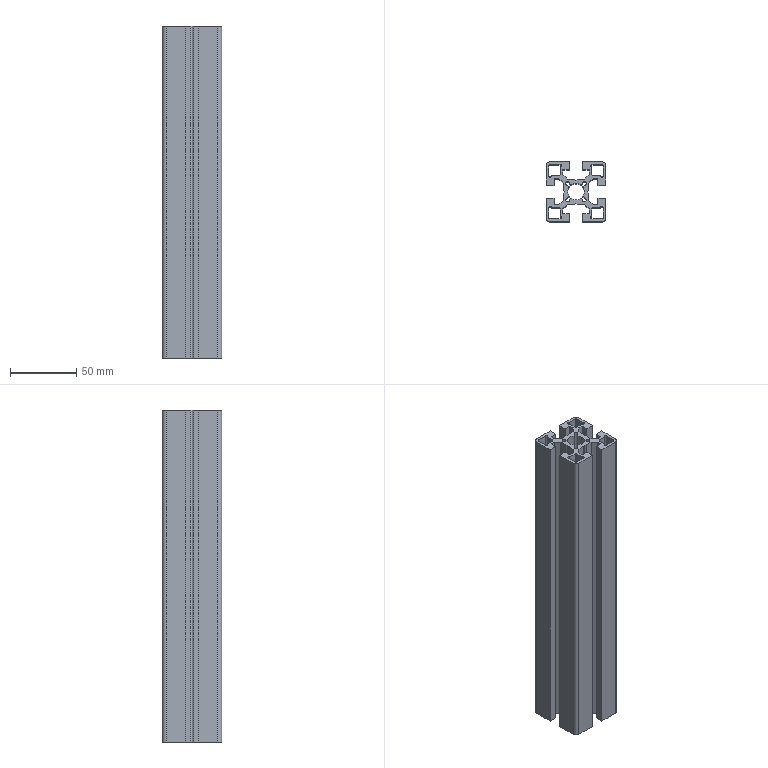Component | SolidWorks | HFS8_4545_08-B-3 | 1 solid | 131 faces | box 45 x 45 x 250 mm | volume 200550 mm3 | plane 82 | cylinder 49 | commonest cylinder face diameters 2 x18 3 x12 1 x10 12.5 x5 6 x4 | material 6061-T6 (SS)
build123d program:
from build123d import *

# Parameters (mm, degrees)
BOSS_EXTRUDE1_DEPTH = 250


with BuildPart() as part:
    # Sketch1 → Boss-Extrude1 (new body)
    with BuildSketch(Plane.XY):
        with BuildLine():
            Line((-19.5, -22.5), (-5, -22.5))
            Line((-5, -22.5), (-5, -16.5))
            Line((-5, -16.5), (-10, -16.5))
            Line((-10, -16.5), (-10, -13))
            Line((-10, -13), (-6.5, -9.5))
            Line((-6.5, -9.5), (-1.212, -9.5))
            Line((-1.212, -9.5), (0, -8.8))
            Line((0, -8.8), (1.212, -9.5))
            Line((1.212, -9.5), (6.5, -9.5))
            Line((6.5, -9.5), (10, -13))
            Line((10, -13), (10, -16.5))
            Line((10, -16.5), (5, -16.5))
            Line((5, -16.5), (5, -22.5))
            Line((5, -22.5), (19.5, -22.5))
            ThreePointArc((19.5, -22.5), (21.621, -21.621), (22.5, -19.5))
            Line((22.5, -19.5), (22.5, -5))
            Line((22.5, -5), (16.5, -5))
            Line((16.5, -5), (16.5, -10))
            Line((16.5, -10), (13, -10))
            Line((13, -10), (9.5, -6.5))
            Line((9.5, -6.5), (9.5, -1.212))
            Line((9.5, -1.212), (8.8, 0))
            Line((8.8, 0), (9.5, 1.212))
            Line((9.5, 1.212), (9.5, 6.5))
            Line((9.5, 6.5), (13, 10))
            Line((13, 10), (16.5, 10))
            Line((16.5, 10), (16.5, 5))
            Line((16.5, 5), (22.5, 5))
            Line((22.5, 5), (22.5, 19.5))
            ThreePointArc((22.5, 19.5), (21.621, 21.621), (19.5, 22.5))
            Line((19.5, 22.5), (5, 22.5))
            Line((5, 22.5), (5, 16.5))
            Line((5, 16.5), (10, 16.5))
            Line((10, 16.5), (10, 13))
            Line((10, 13), (6.5, 9.5))
            Line((6.5, 9.5), (1.212, 9.5))
            Line((1.212, 9.5), (0, 8.8))
            Line((0, 8.8), (-1.212, 9.5))
            Line((-1.212, 9.5), (-6.5, 9.5))
            Line((-6.5, 9.5), (-10, 13))
            Line((-10, 13), (-10, 16.5))
            Line((-10, 16.5), (-5, 16.5))
            Line((-5, 16.5), (-5, 22.5))
            Line((-5, 22.5), (-19.5, 22.5))
            ThreePointArc((-19.5, 22.5), (-21.621, 21.621), (-22.5, 19.5))
            Line((-22.5, 19.5), (-22.5, 5))
            Line((-22.5, 5), (-16.5, 5))
            Line((-16.5, 5), (-16.5, 10))
            Line((-16.5, 10), (-13, 10))
            Line((-13, 10), (-9.5, 6.5))
            Line((-9.5, 6.5), (-9.5, 1.212))
            Line((-9.5, 1.212), (-8.8, 0))
            Line((-8.8, 0), (-9.5, -1.212))
            Line((-9.5, -1.212), (-9.5, -6.5))
            Line((-9.5, -6.5), (-13, -10))
            Line((-13, -10), (-16.5, -10))
            Line((-16.5, -10), (-16.5, -5))
            Line((-16.5, -5), (-22.5, -5))
            Line((-22.5, -5), (-22.5, -19.5))
            ThreePointArc((-22.5, -19.5), (-21.621, -21.621), (-19.5, -22.5))
        make_face()
        with BuildLine():
            Line((12, 18.5), (12, 13))
            ThreePointArc((12, 13), (12.293, 12.293), (13, 12))
            Line((13, 12), (18.5, 12))
            ThreePointArc((18.5, 12), (19.5, 11), (20.5, 12))
            Line((20.5, 12), (20.5, 19.5))
            ThreePointArc((20.5, 19.5), (20.207, 20.207), (19.5, 20.5))
            Line((19.5, 20.5), (12, 20.5))
            ThreePointArc((12, 20.5), (11, 19.5), (12, 18.5))
        make_face(mode=Mode.SUBTRACT)
        with BuildLine():
            Line((12, -20.5), (19.5, -20.5))
            ThreePointArc((19.5, -20.5), (20.207, -20.207), (20.5, -19.5))
            Line((20.5, -19.5), (20.5, -12))
            ThreePointArc((20.5, -12), (19.5, -11), (18.5, -12))
            Line((18.5, -12), (13, -12))
            ThreePointArc((13, -12), (12.293, -12.293), (12, -13))
            Line((12, -13), (12, -18.5))
            ThreePointArc((12, -18.5), (11, -19.5), (12, -20.5))
        make_face(mode=Mode.SUBTRACT)
        with BuildLine():
            Line((-4.725, -6.139), (-3.947, -5.361))
            ThreePointArc((-3.947, -5.361), (-3.649, -5.217), (-3.327, -5.291))
            ThreePointArc((-3.327, -5.291), (0, -6.25), (3.327, -5.291))
            ThreePointArc((3.327, -5.291), (3.649, -5.217), (3.947, -5.361))
            Line((3.947, -5.361), (4.725, -6.139))
            ThreePointArc((4.725, -6.139), (7.283, -7.283), (6.139, -4.725))
            Line((6.139, -4.725), (5.361, -3.947))
            ThreePointArc((5.361, -3.947), (5.217, -3.649), (5.291, -3.327))
            ThreePointArc((5.291, -3.327), (6.25, 0), (5.291, 3.327))
            ThreePointArc((5.291, 3.327), (5.217, 3.649), (5.361, 3.947))
            Line((5.361, 3.947), (6.139, 4.725))
            ThreePointArc((6.139, 4.725), (7.283, 7.283), (4.725, 6.139))
            Line((4.725, 6.139), (3.947, 5.361))
            ThreePointArc((3.947, 5.361), (3.649, 5.217), (3.327, 5.291))
            ThreePointArc((3.327, 5.291), (0, 6.25), (-3.327, 5.291))
            ThreePointArc((-3.327, 5.291), (-3.649, 5.217), (-3.947, 5.361))
            Line((-3.947, 5.361), (-4.725, 6.139))
            ThreePointArc((-4.725, 6.139), (-7.283, 7.283), (-6.139, 4.725))
            Line((-6.139, 4.725), (-5.361, 3.947))
            ThreePointArc((-5.361, 3.947), (-5.217, 3.649), (-5.291, 3.327))
            ThreePointArc((-5.291, 3.327), (-6.25, 0), (-5.291, -3.327))
            ThreePointArc((-5.291, -3.327), (-5.217, -3.649), (-5.361, -3.947))
            Line((-5.361, -3.947), (-6.139, -4.725))
            ThreePointArc((-6.139, -4.725), (-7.283, -7.283), (-4.725, -6.139))
        make_face(mode=Mode.SUBTRACT)
        with BuildLine():
            Line((-19.5, -20.5), (-12, -20.5))
            ThreePointArc((-12, -20.5), (-11, -19.5), (-12, -18.5))
            Line((-12, -18.5), (-12, -13))
            ThreePointArc((-12, -13), (-12.293, -12.293), (-13, -12))
            Line((-13, -12), (-18.5, -12))
            ThreePointArc((-18.5, -12), (-19.5, -11), (-20.5, -12))
            Line((-20.5, -12), (-20.5, -19.5))
            ThreePointArc((-20.5, -19.5), (-20.207, -20.207), (-19.5, -20.5))
        make_face(mode=Mode.SUBTRACT)
        with BuildLine():
            Line((-18.5, 12), (-13, 12))
            ThreePointArc((-13, 12), (-12.293, 12.293), (-12, 13))
            Line((-12, 13), (-12, 18.5))
            ThreePointArc((-12, 18.5), (-11, 19.5), (-12, 20.5))
            Line((-12, 20.5), (-19.5, 20.5))
            ThreePointArc((-19.5, 20.5), (-20.207, 20.207), (-20.5, 19.5))
            Line((-20.5, 19.5), (-20.5, 12))
            ThreePointArc((-20.5, 12), (-19.5, 11), (-18.5, 12))
        make_face(mode=Mode.SUBTRACT)
    extrude(amount=-BOSS_EXTRUDE1_DEPTH)


solid = part.part

# Placed as in the assembly
solid = solid.moved(Location((-65.506, -351.913, -947.928), (0, 0, 0)))